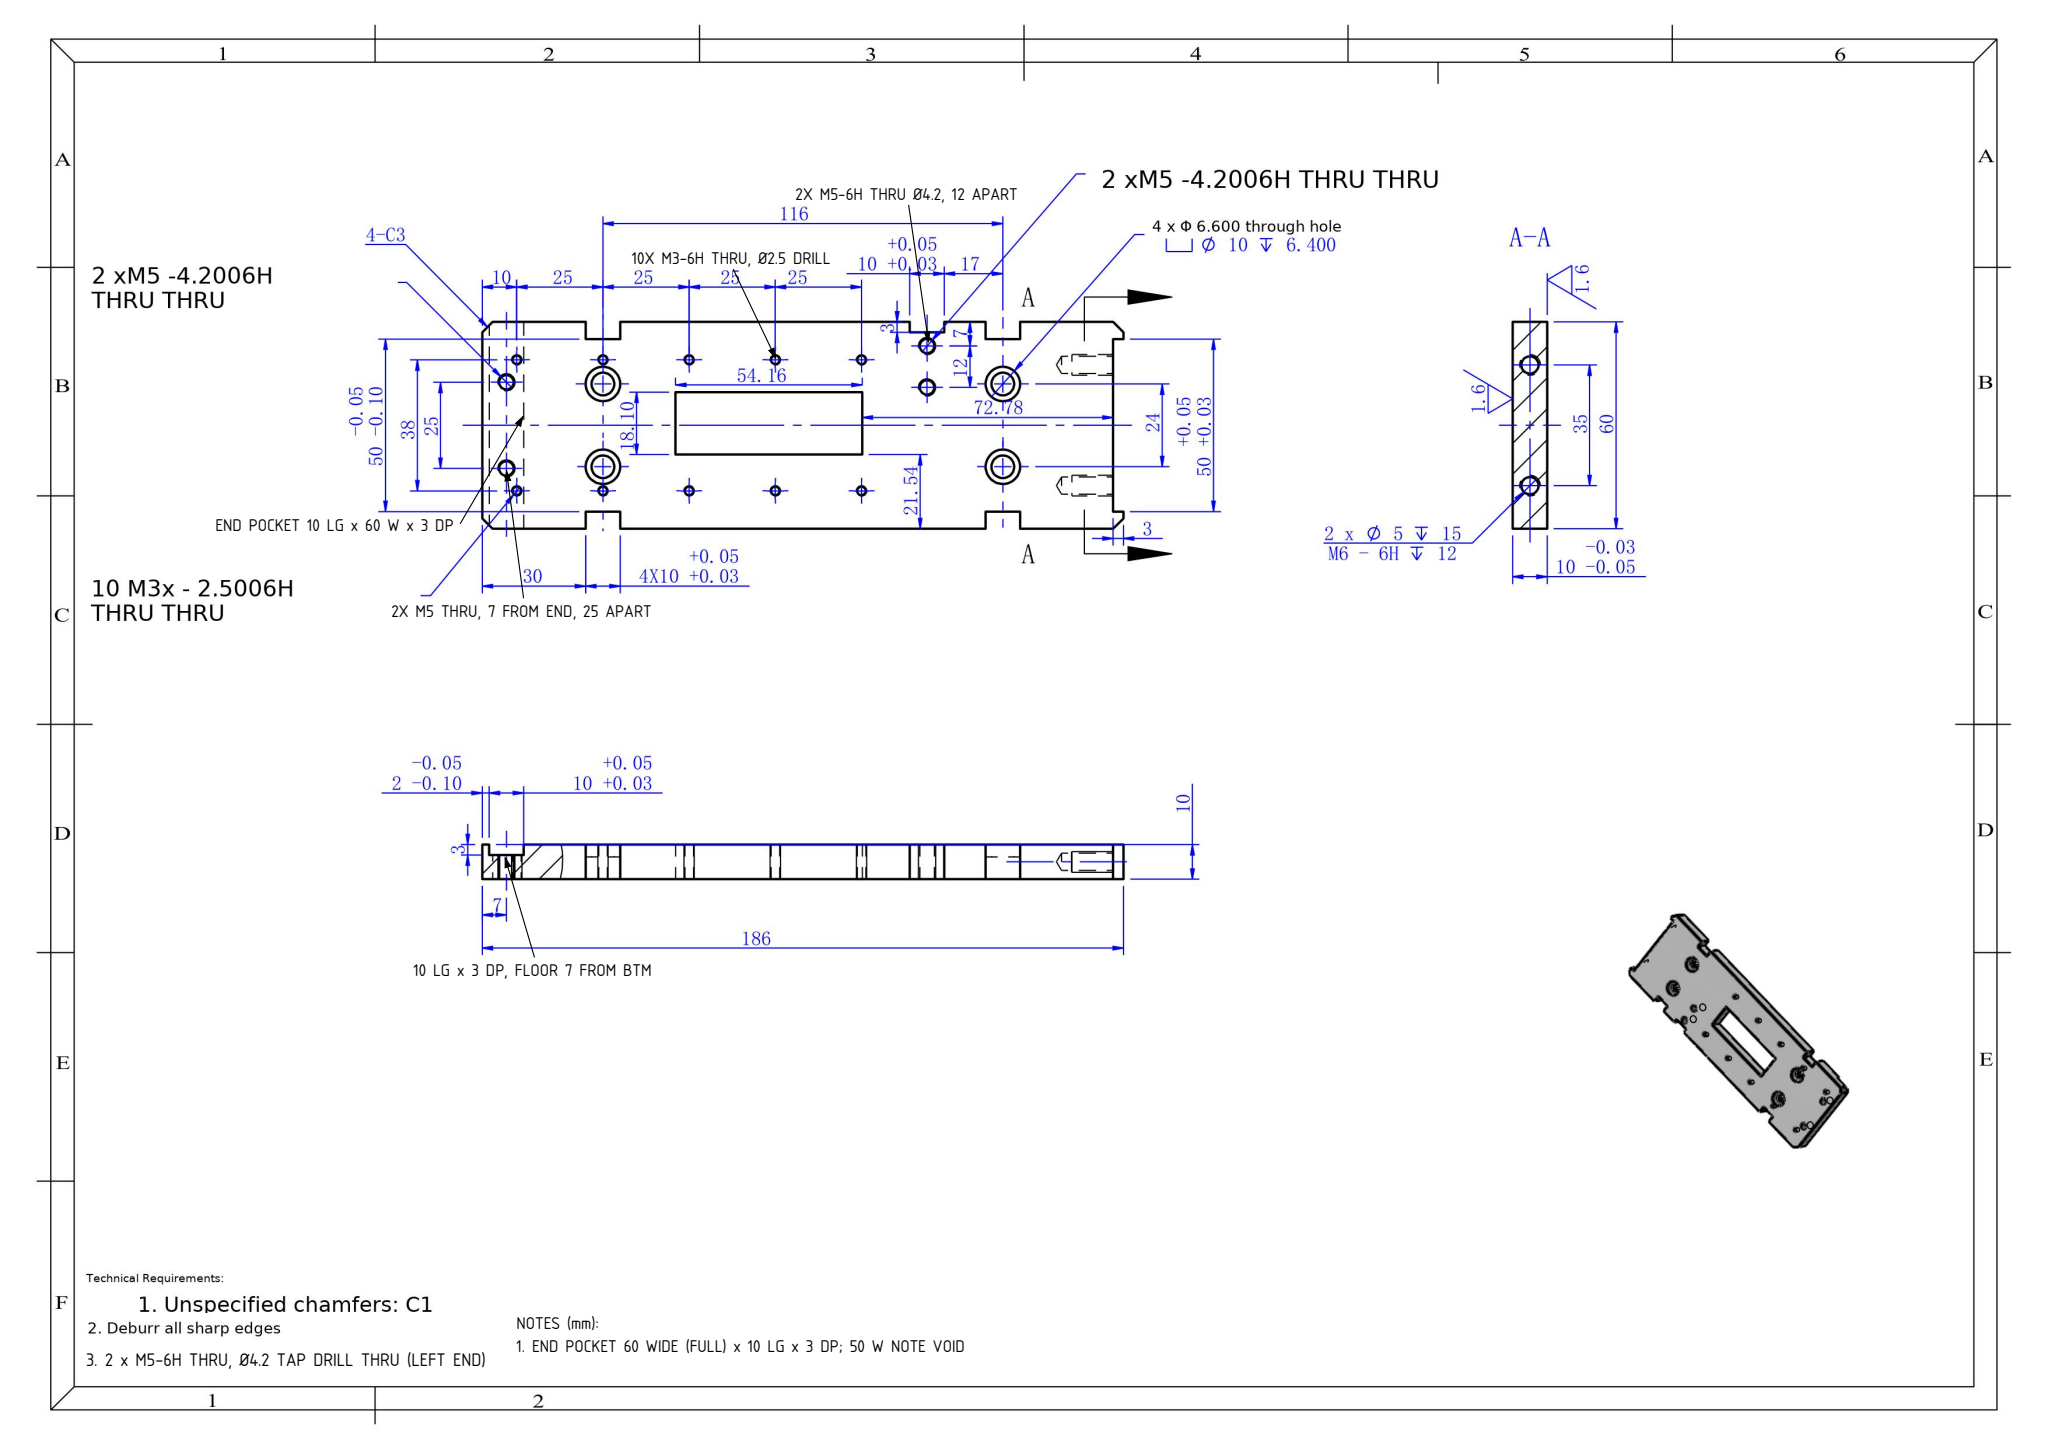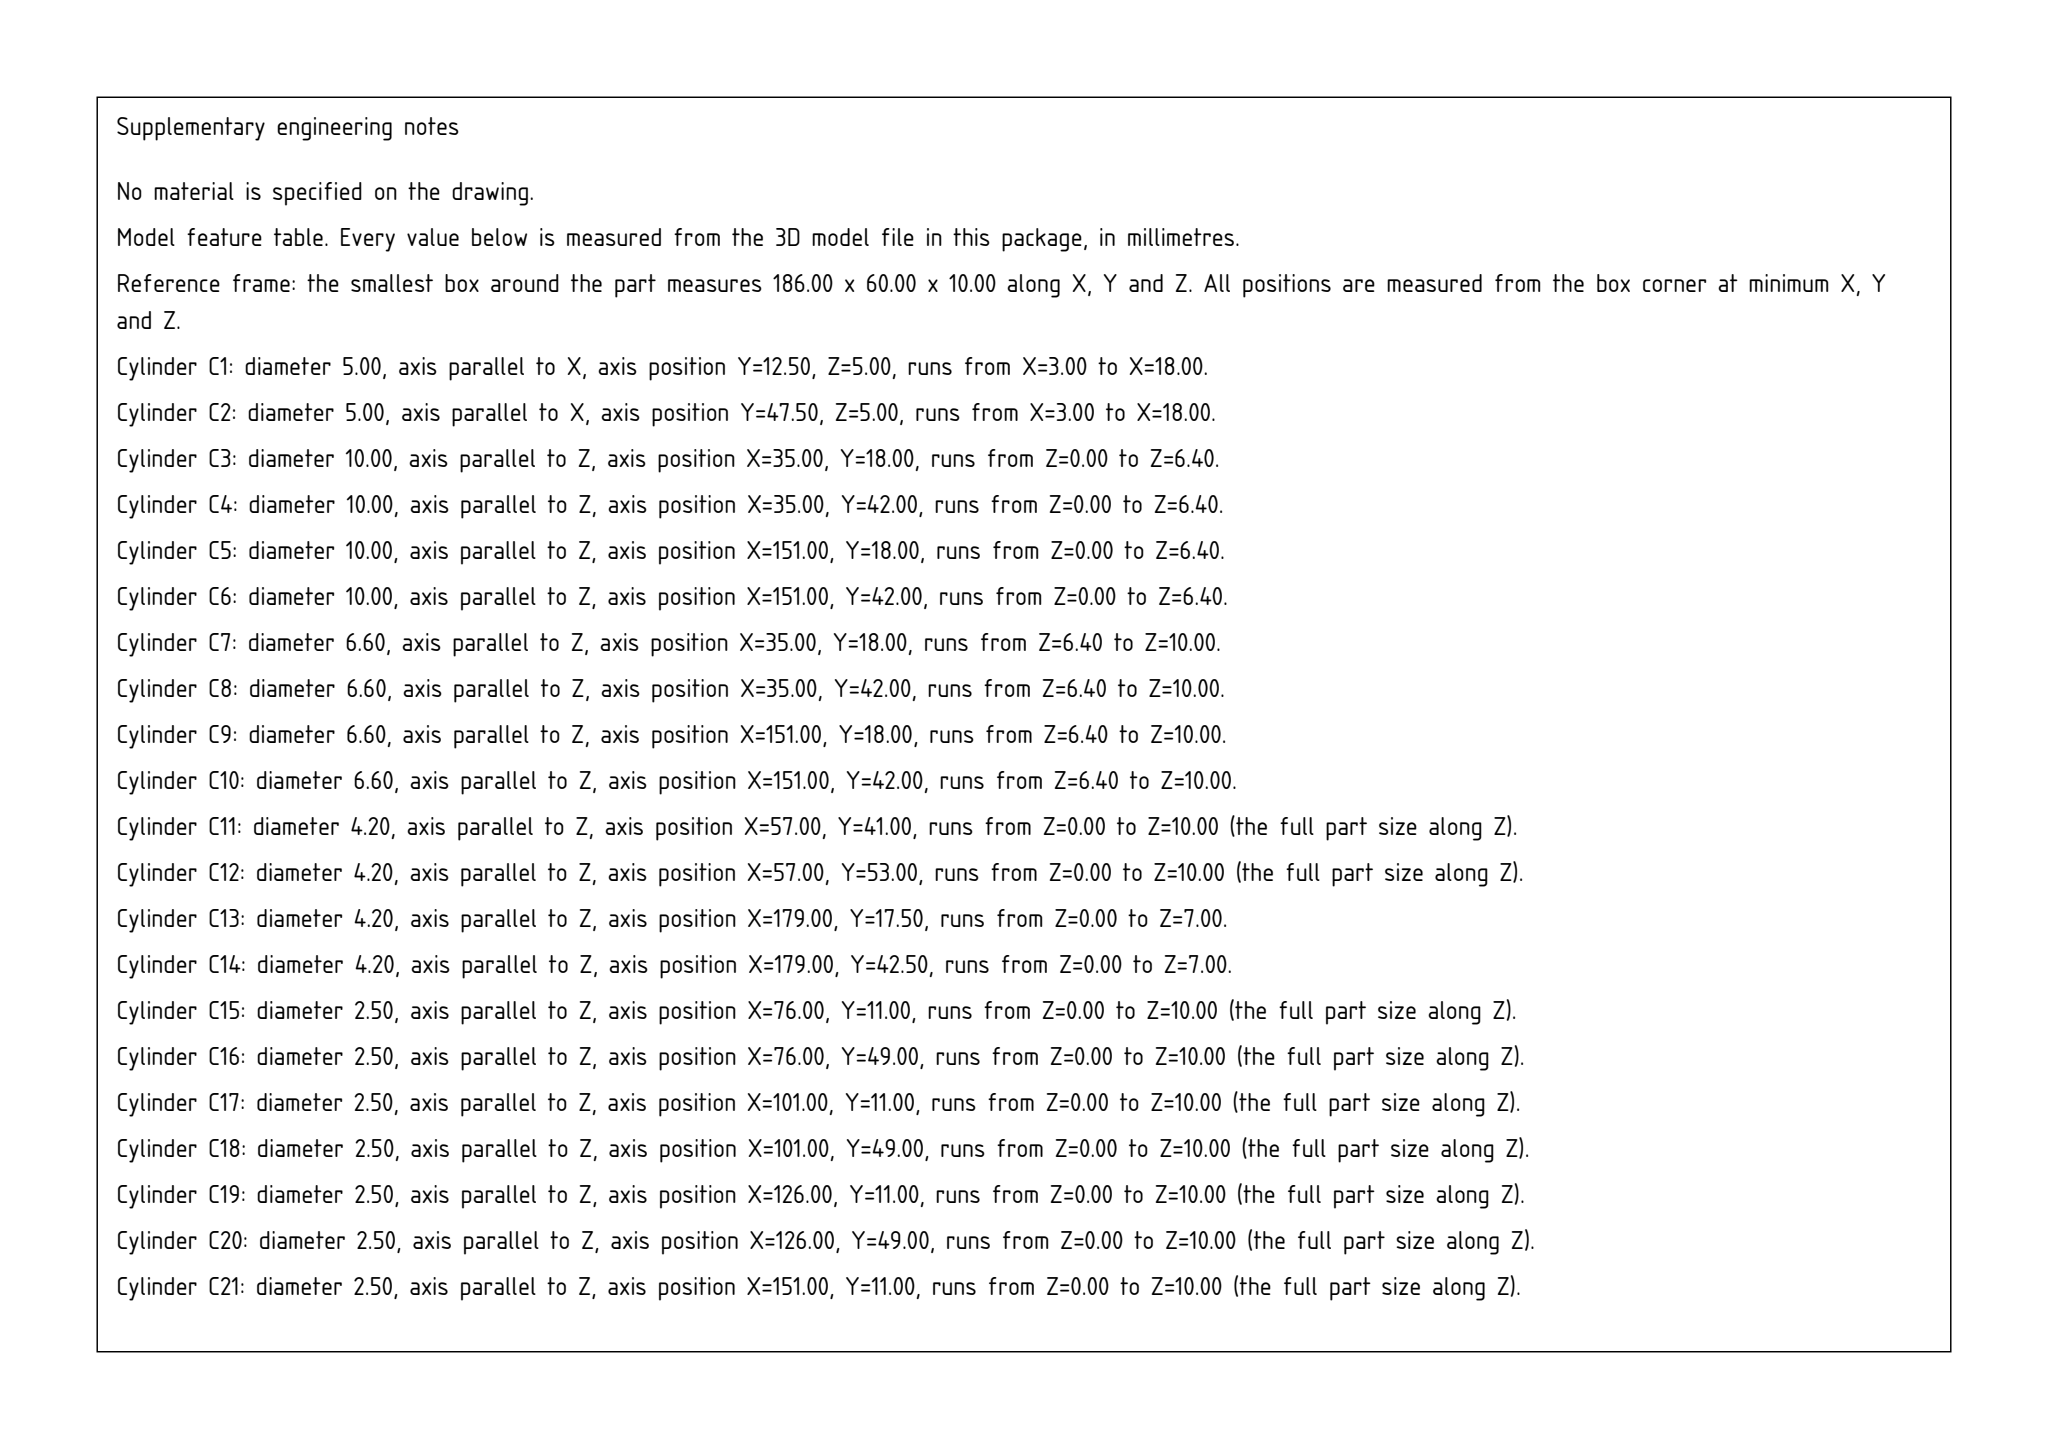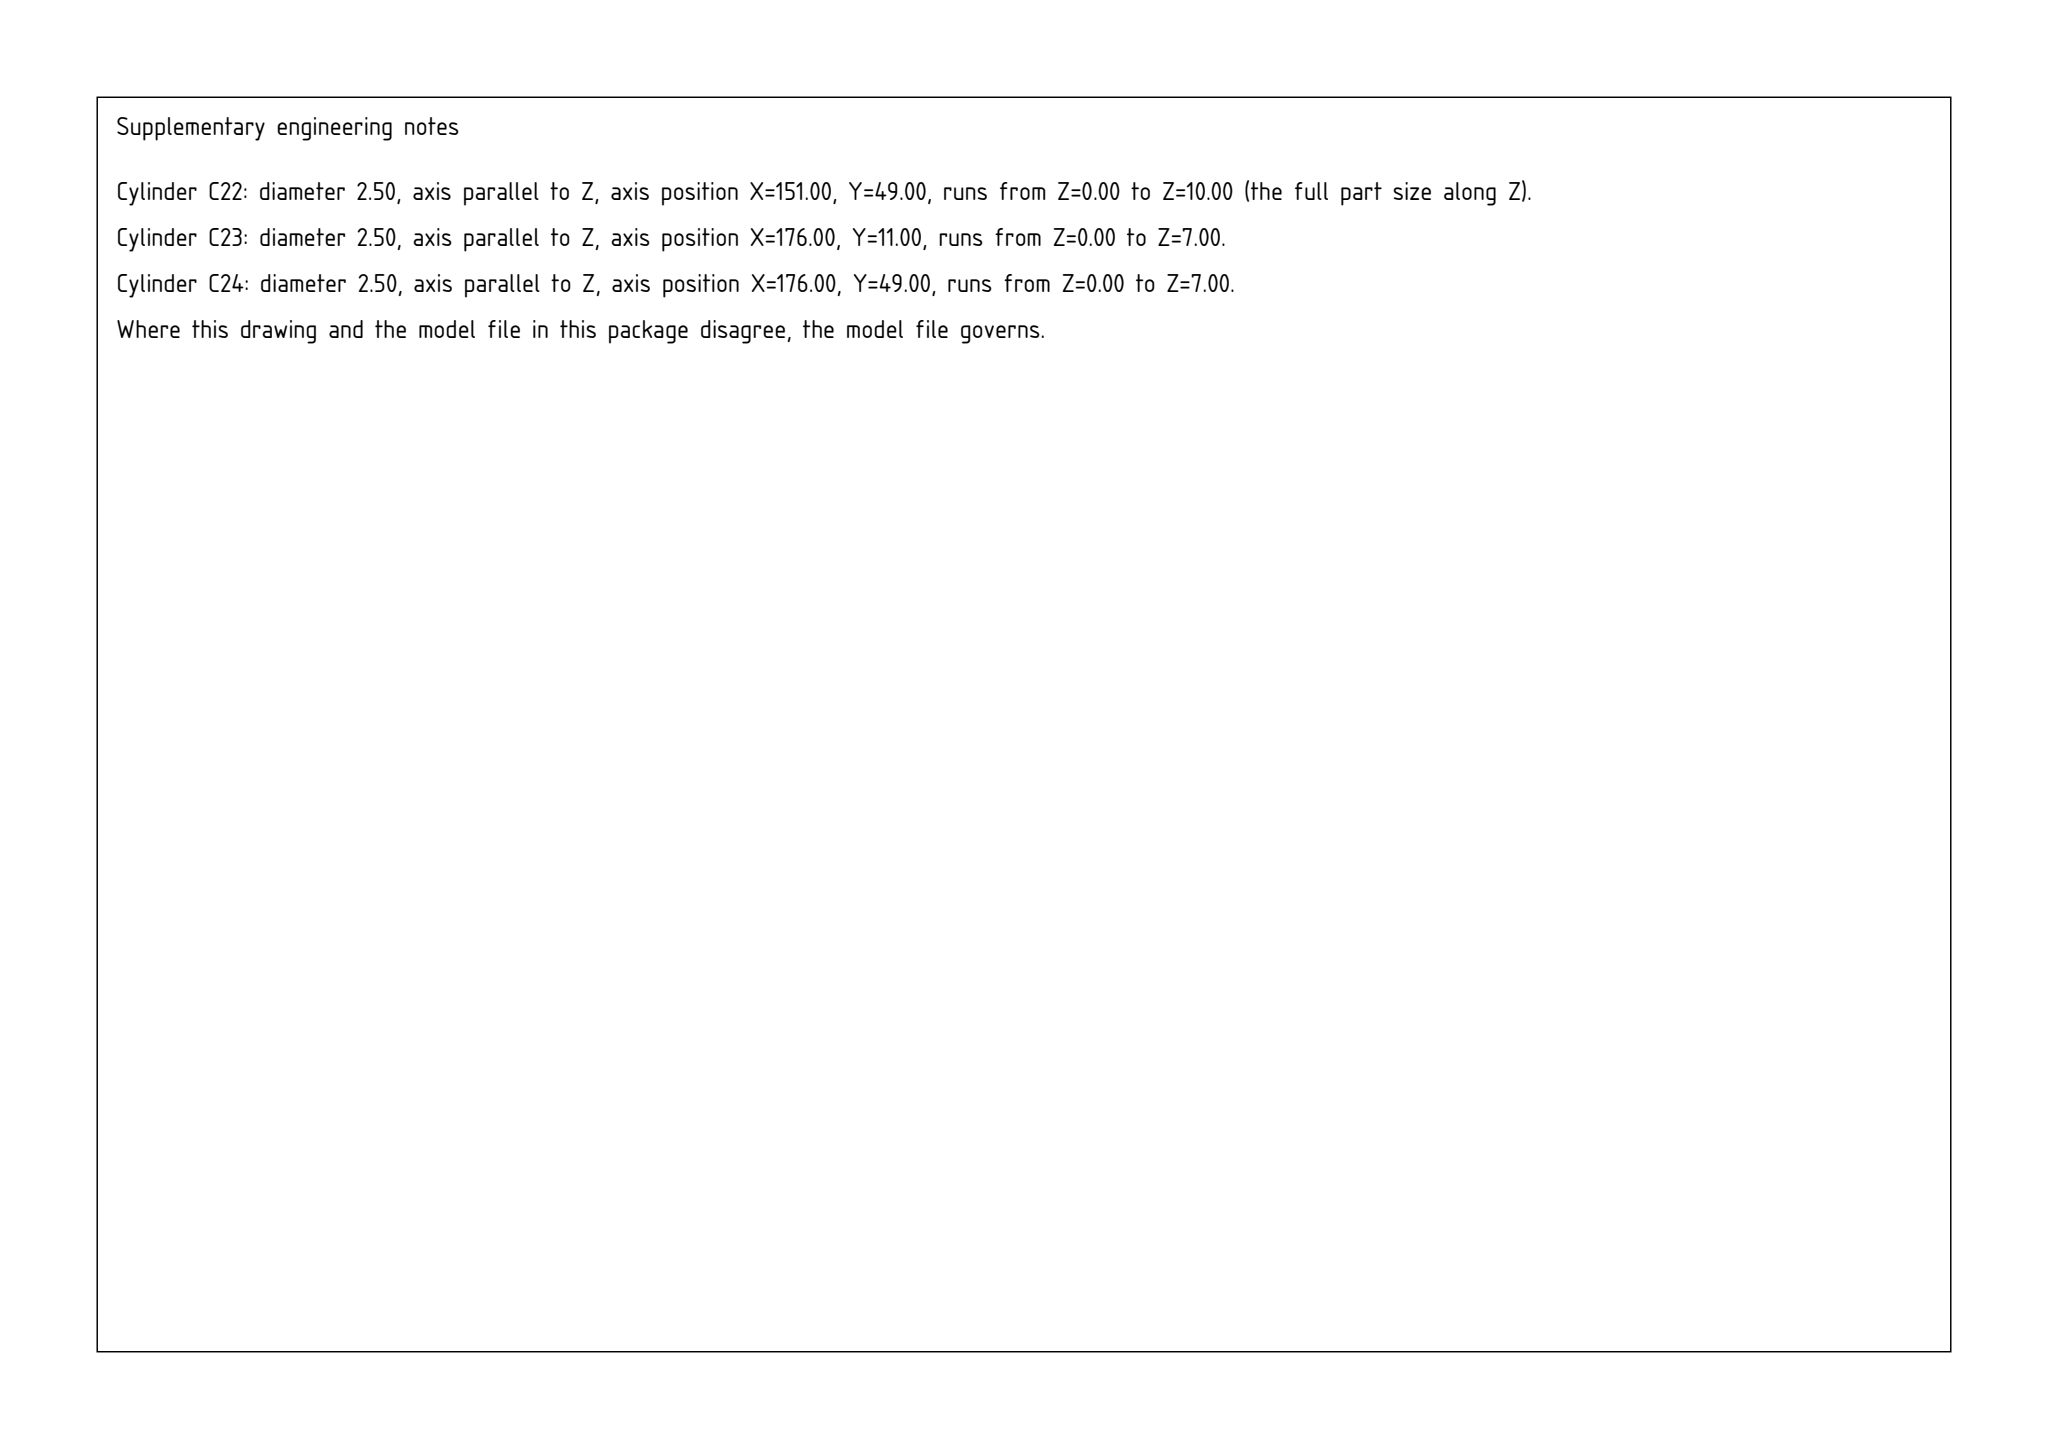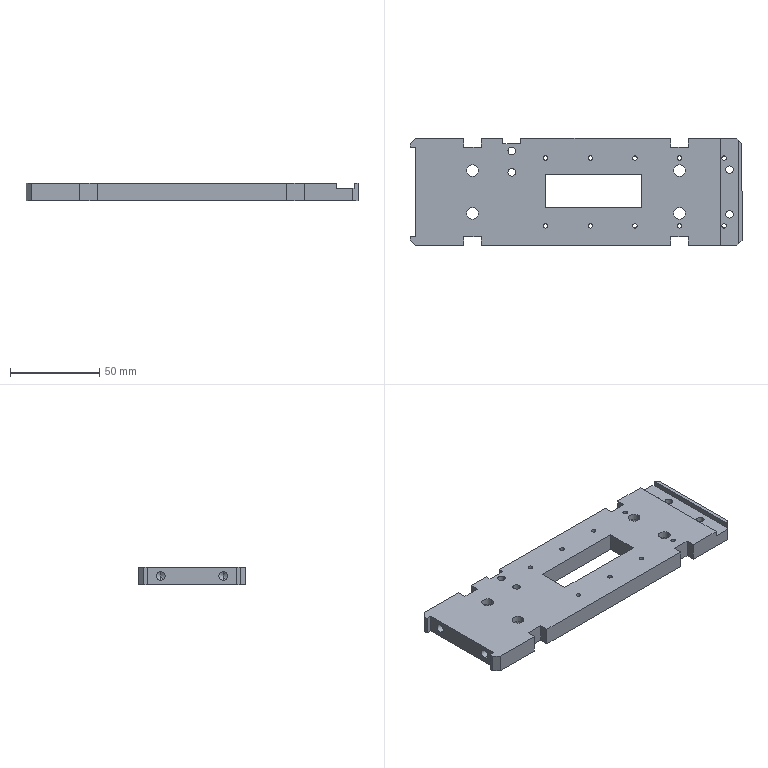Part | SolidWorks | mm | 1 solid | 98 faces | box 186 x 60 x 10 mm | volume 91974 mm3 | cylinder 48 | plane 46 | cone 4 | commonest cylinder face diameters 2.5 x20 4.2 x8 10 x8 6.6 x8 5 x4
Drawing notes:
END POCKET: 60 WIDE (FULL) x 10 LG x 3 DP, FLOOR 7 FROM BTM | from the solid: Plane z=7 extent x[174,184] y[0,60]; face x=174 z[7,10]; face x=184 z[7,10]; top z=10 ends at x=174
2 x M5 THRU: 7 FROM LEFT END FACE, 25 APART, SYM ABT HORIZ C/L | from the solid: Ø4.2 z-holes at (179,17.5) & (179,42.5); bbox X=186 so 186-179=7 from end face; 42.5-17.5=25, sym about Y=30 of 60 wide
END POCKET: 10 LG x 60 WIDE (FULL) x 3 DP | from the solid: z=7.0 plane, x[174,184], y[0,60], area 561; top face z=10 ends at x=174 -> 10 long x 60 wide x 3 deep step
2 x M5-6H THRU, Ø4.2 TAP DRILL THRU (LEFT END) | from the solid: Ø4.2 z-holes at (179,17.5),(179,42.5) from z=0 to 7 = full local thk (pocket floor z=7)
2 x M5-6H THRU, Ø4.2 DRILL THRU (NOTCH PAIR, 12 APART) | from the solid: Ø4.2 z-holes at (57,41),(57,53) from z=0 to 10 = full 10 thk; 53-41=12, y=53 is 7 from y=60 edge
10 x M3-6H THRU, Ø2.5 TAP DRILL THRU | from the solid: Ø2.5 z-holes at x=76,101,126,151 (y=11 & 49) z0-10 and x=176 (y=11 & 49) z0-7 = thru local thk; 10 places
END POCKET 60 WIDE (FULL) x 10 LG x 3 DP; 50 W NOTE VOID | from the solid: Pocket floor z=7 spans y[0,60] full width, x[174,184] = 10 long, depth 10-7=3; no 50 wide face exists
build123d program:
from build123d import *

# Parameters (mm, degrees)
SKETCH1_W                                       = 186
SKETCH1_H                                       = 60
BOSS_EXTRUDE1_DEPTH                             = 10
SKETCH2_W                                       = 10
SKETCH2_H                                       = 5
CUT_EXTRUDE1_DEPTH                              = 144.377
SKETCH3_W                                       = 3
SKETCH3_H                                       = 50
CUT_EXTRUDE2_DEPTH                              = 144.377
M6_TAPPED_HOLE1_D                               = 5
M6_TAPPED_HOLE1_DEPTH                           = 15
M6_TAPPED_HOLE1_TIP                             = 1.502
SKETCH6_W                                       = 10
SKETCH6_H                                       = 3
CUT_EXTRUDE3_DEPTH                              = 144.377
CHAMFER1_SIZE                                   = 3
SKETCH7_W                                       = 10
SKETCH7_H                                       = 3
CUT_EXTRUDE4_DEPTH                              = 147.425
M6_HEX_SOCKET_HEAD_CAP_SCREW_CBORE1_D           = 6.6
M6_HEX_SOCKET_HEAD_CAP_SCREW_CBORE1_CBORE_D     = 10
M6_HEX_SOCKET_HEAD_CAP_SCREW_CBORE1_CBORE_DEPTH = 6.4
M5_TAPPED_HOLE1_D                               = 4.2
M3_TAPPED_HOLE1_D                               = 2.5
M5_TAPPED_HOLE2_D                               = 4.2
SKETCH17_W                                      = 54.161
SKETCH17_H                                      = 18.103
CUT_EXTRUDE5_DEPTH                              = 35


with BuildPart() as part:
    # Sketch1 → Boss-Extrude1 (new body)
    with BuildSketch(Plane.XY):
        with Locations((40.192, 22.124)):
            Rectangle(SKETCH1_W, SKETCH1_H)
    extrude(amount=BOSS_EXTRUDE1_DEPTH)

    # Sketch2 → Cut-Extrude1 (cut, through all)
    with BuildSketch(Plane(origin=(0, 0, 0), x_dir=(-1, 0, 0), z_dir=(0, 0, -1))):
        with Locations((17.808, 49.624)):
            Rectangle(SKETCH2_W, SKETCH2_H)
        with Locations((17.808, -5.376)):
            Rectangle(SKETCH2_W, SKETCH2_H)
    cut_extrude1 = extrude(amount=-CUT_EXTRUDE1_DEPTH, mode=Mode.SUBTRACT)

    # Mirror1: Cut-Extrude1 across plane
    add(cut_extrude1.mirror(Plane(origin=(40.192, 0, 0), x_dir=(0, 0, 1), z_dir=(1, 0, 0))), mode=Mode.SUBTRACT)

    # Sketch3 → Cut-Extrude2 (cut, through all)
    with BuildSketch(Plane.XY.offset(10)):
        with Locations((-51.308, 22.124)):
            Rectangle(SKETCH3_W, SKETCH3_H)
    extrude(amount=-CUT_EXTRUDE2_DEPTH, mode=Mode.SUBTRACT)

    # M6 Tapped Hole1
    with Locations(Plane.ZY.offset(49.808)):
        with Locations((5, 39.624), (5, 4.624)):
            Hole(M6_TAPPED_HOLE1_D / 2, depth=M6_TAPPED_HOLE1_DEPTH)
            with Locations((0, 0, -(M6_TAPPED_HOLE1_DEPTH + M6_TAPPED_HOLE1_TIP / 2))):  # 118° drill point
                Cone(0, M6_TAPPED_HOLE1_D / 2, M6_TAPPED_HOLE1_TIP, mode=Mode.SUBTRACT)

    # Sketch6 → Cut-Extrude3 (cut, through all)
    with BuildSketch(Plane(origin=(0, 0, 0), x_dir=(-1, 0, 0), z_dir=(0, 0, -1))):
        with Locations((-4.192, 50.624)):
            Rectangle(SKETCH6_W, SKETCH6_H)
    extrude(amount=-CUT_EXTRUDE3_DEPTH, mode=Mode.SUBTRACT)

    # Chamfer1
    chamfer1_edges = [part.edges().sort_by_distance(p)[0] for p in [
        (133.192, -7.876, 5),
        (-52.808, -7.876, 5),
        (-52.808, 52.124, 5),
        (133.192, 52.124, 5),
    ]]
    chamfer(chamfer1_edges, length=CHAMFER1_SIZE)

    # Sketch7 → Cut-Extrude4 (cut, through all)
    with BuildSketch(Plane(origin=(0, 52.124, 0), x_dir=(1, 0, 0), z_dir=(0, 1, 0))):
        with Locations((126.192, -8.5)):
            Rectangle(SKETCH7_W, SKETCH7_H)
    extrude(amount=-CUT_EXTRUDE4_DEPTH, mode=Mode.SUBTRACT)

    # M6 Hex Socket Head Cap Screw CBORE1 (through all)
    with Locations(Plane(origin=(0, 0, 0), x_dir=(-1, 0, 0), z_dir=(0, 0, -1))):
        with Locations((17.808, 34.124), (17.808, 10.124), (-98.192, 34.124), (-98.192, 10.124)):
            CounterBoreHole(M6_HEX_SOCKET_HEAD_CAP_SCREW_CBORE1_D / 2, M6_HEX_SOCKET_HEAD_CAP_SCREW_CBORE1_CBORE_D / 2, M6_HEX_SOCKET_HEAD_CAP_SCREW_CBORE1_CBORE_DEPTH)

    # M5 Tapped Hole1 (through all)
    with Locations(Plane.XY.offset(10)):
        with Locations((4.192, 45.124), (4.192, 33.124)):
            Hole(M5_TAPPED_HOLE1_D / 2)

    # M3 Tapped Hole1 (through all)
    with Locations(Plane(origin=(0, 0, 0), x_dir=(-1, 0, 0), z_dir=(0, 0, -1))):
        with Locations((-23.192, 41.124), (-48.192, 41.124), (-73.192, 41.124), (-98.192, 41.124), (-123.192, 41.124), (-123.192, 3.124), (-98.192, 3.124), (-73.192, 3.124), (-48.192, 3.124), (-23.192, 3.124)):
            Hole(M3_TAPPED_HOLE1_D / 2)

    # M5 Tapped Hole2 (through all)
    with Locations(Plane.XY.offset(7)):
        with Locations((126.192, 34.624), (126.192, 9.624)):
            Hole(M5_TAPPED_HOLE2_D / 2)

    # Sketch17 → Cut-Extrude5 (cut)
    with BuildSketch(Plane.XY.offset(10)):
        with Locations((50.053, 22.712)):
            Rectangle(SKETCH17_W, SKETCH17_H)
    extrude(amount=-CUT_EXTRUDE5_DEPTH, mode=Mode.SUBTRACT)


solid = part.part